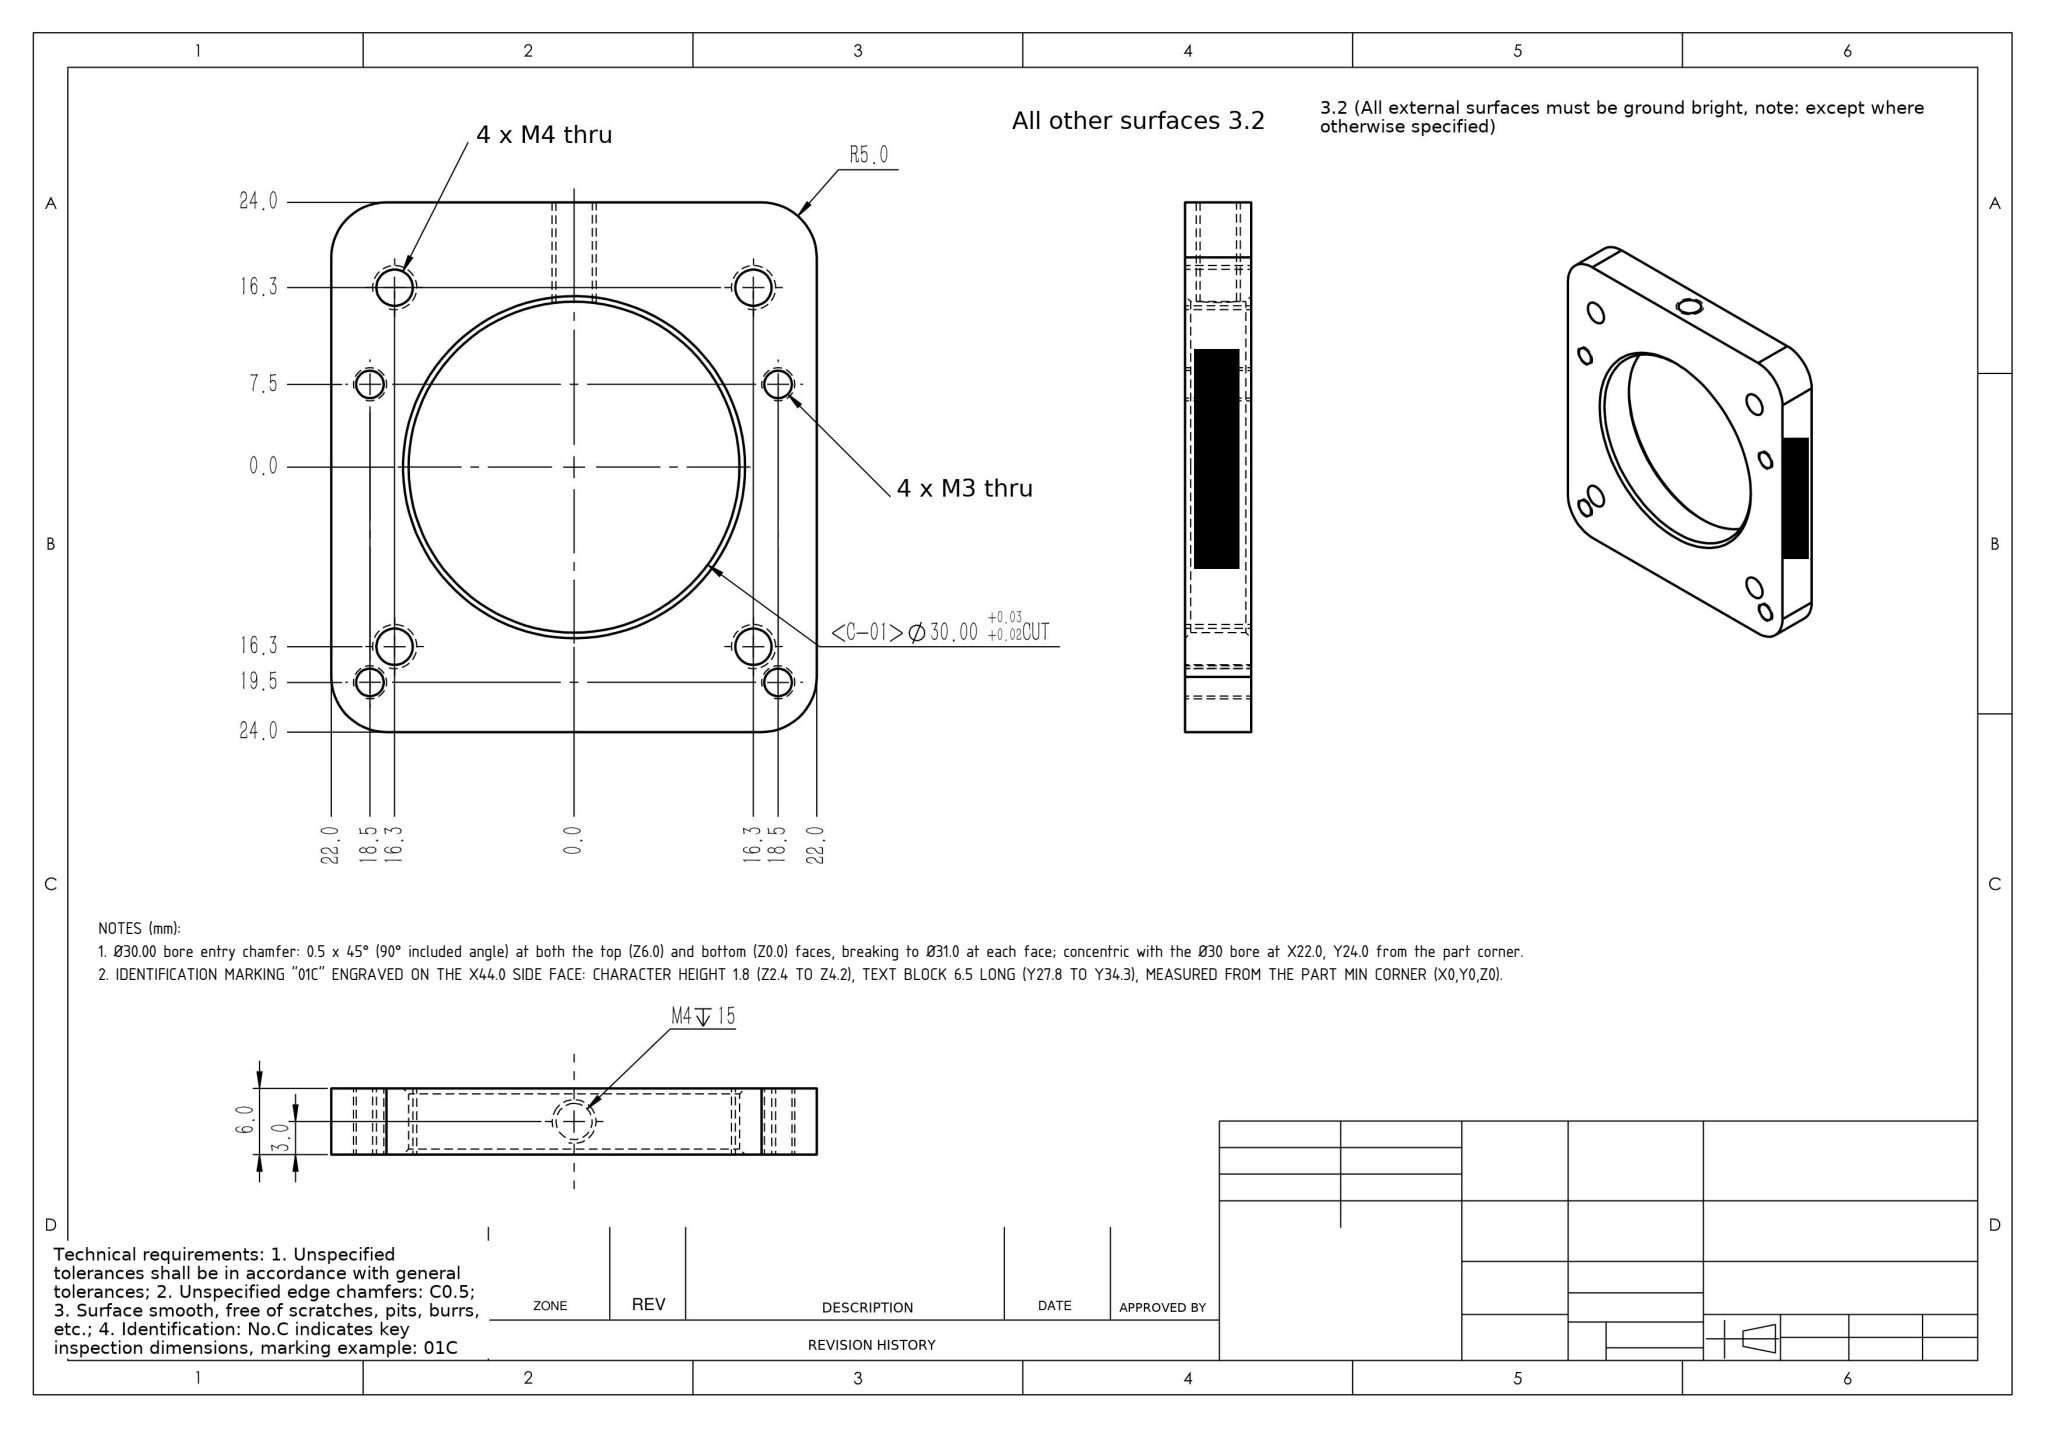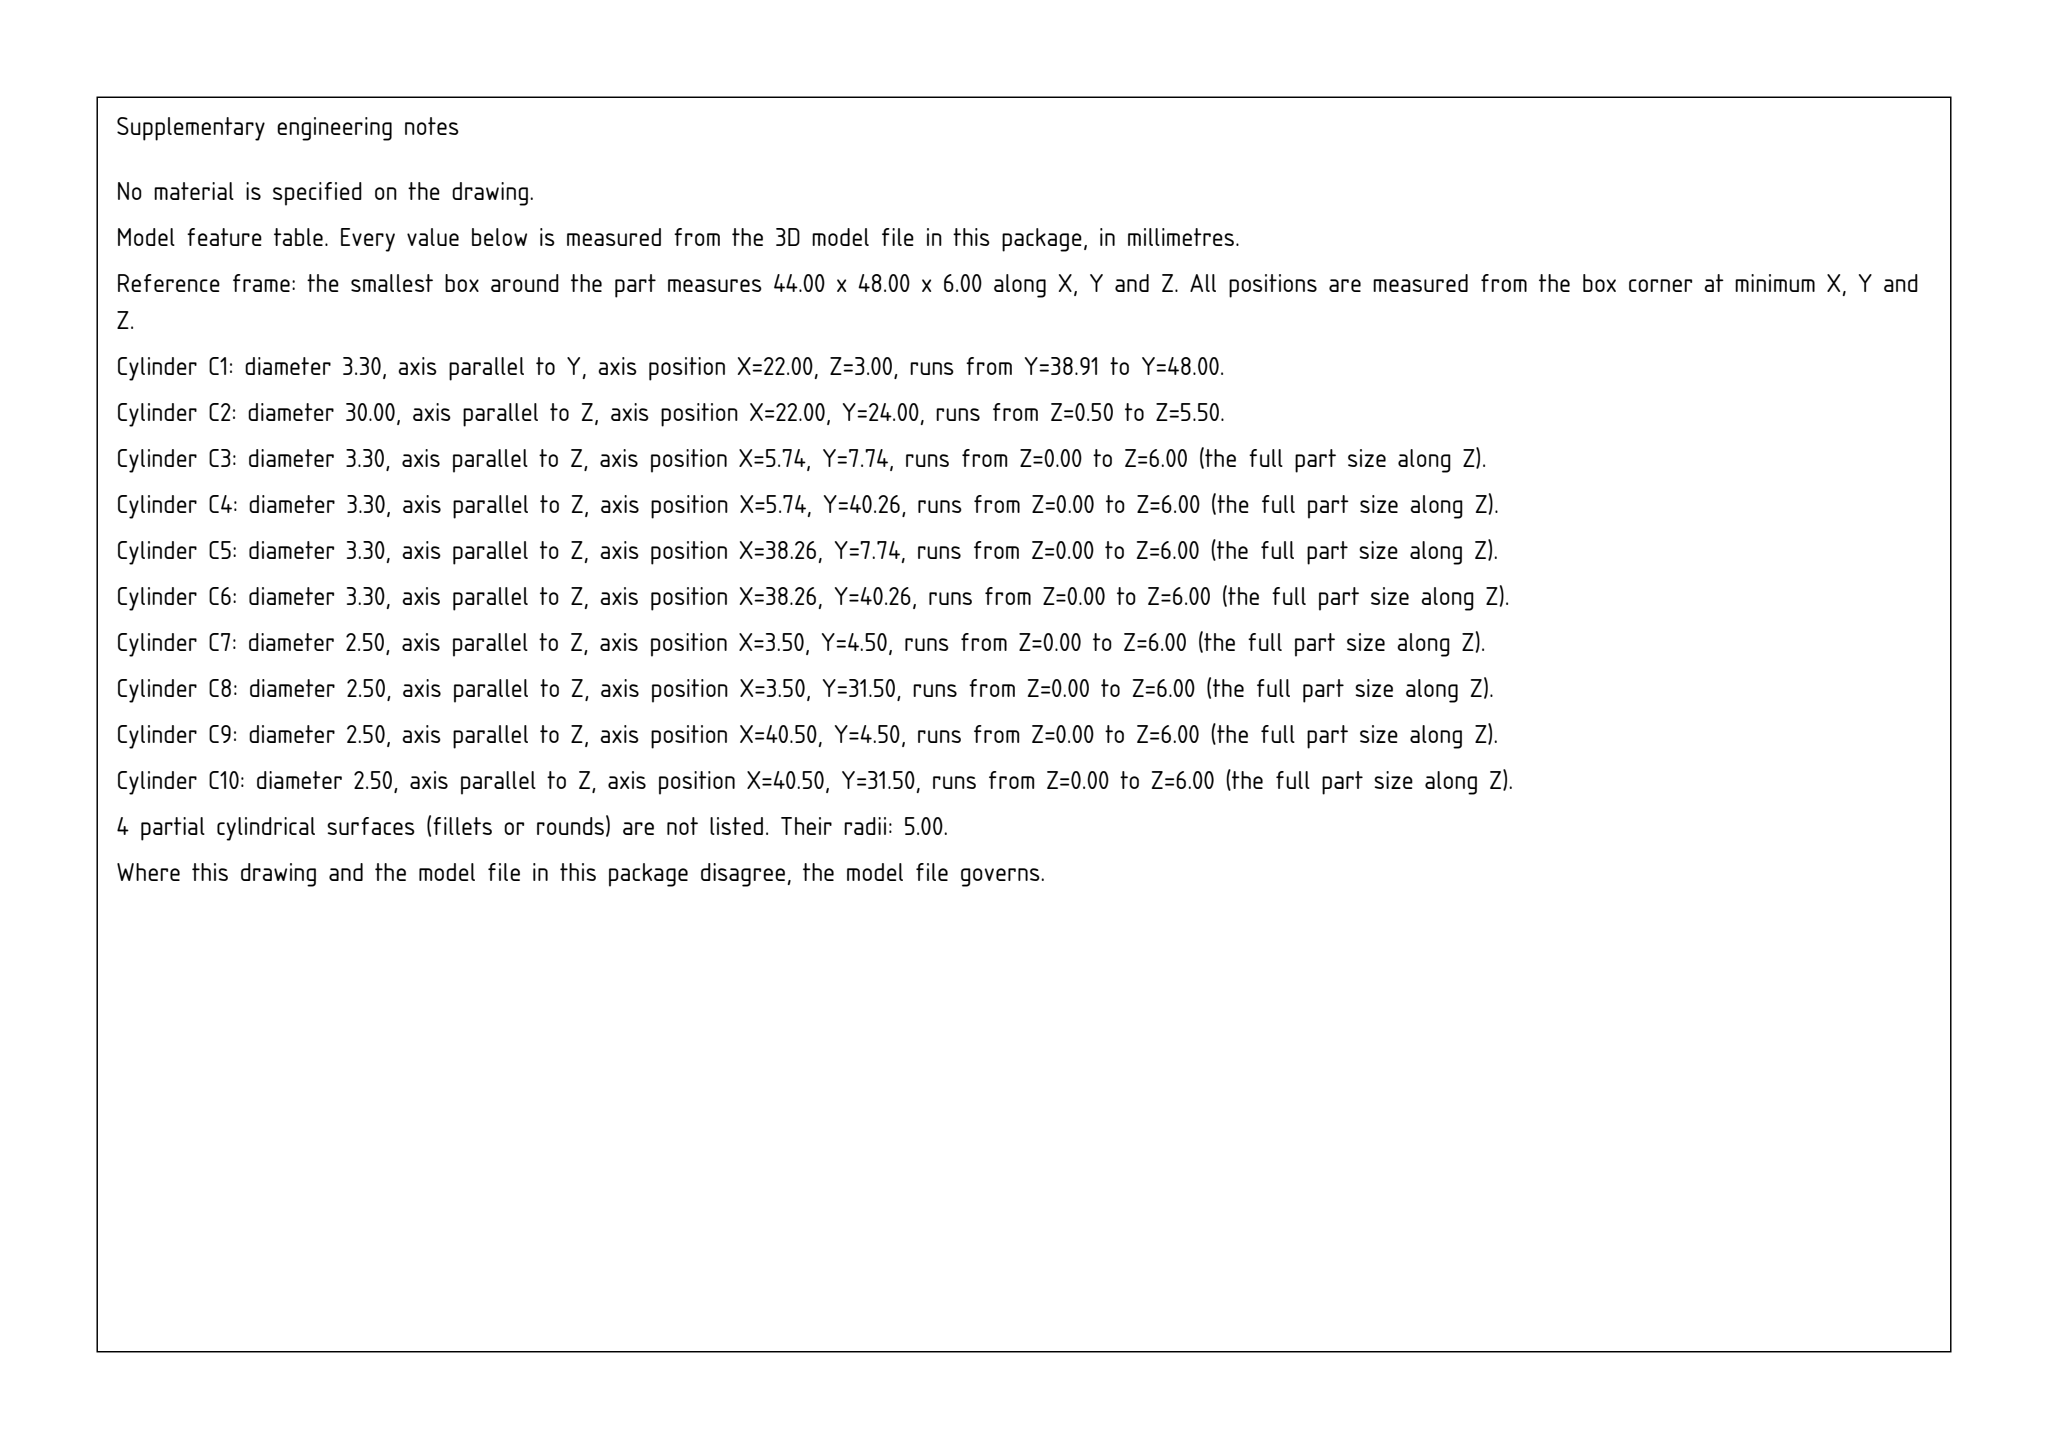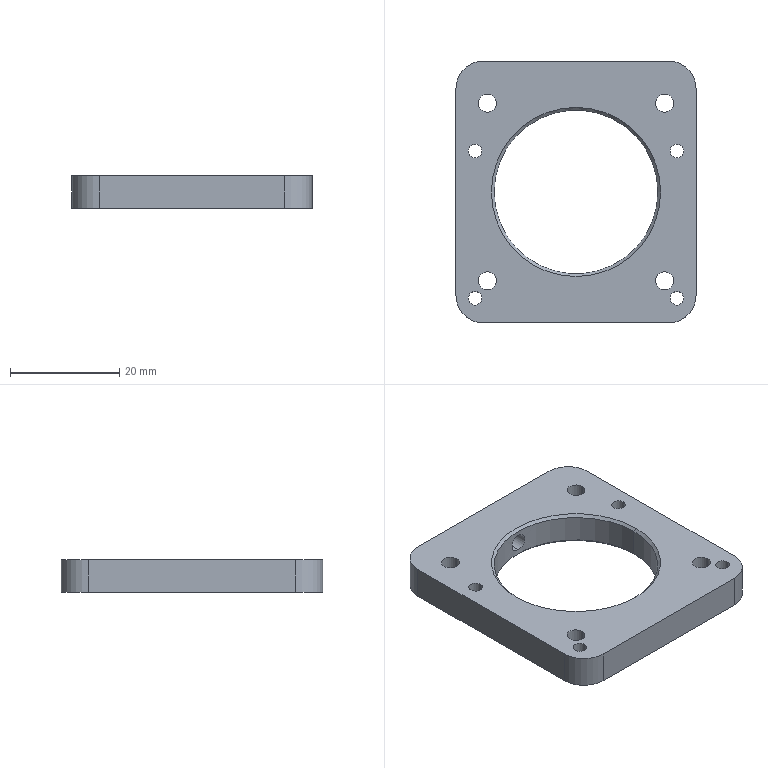Part | SolidWorks | mm | 1 solid | 43 faces | box 44 x 48 x 6 mm | volume 7878 mm3 | cylinder 24 | plane 15 | cone 4 | commonest cylinder face diameters 3.3 x10 2.5 x8 10 x4 30 x2
Drawing notes:
Ø30.00 bore entry chamfer: 0.5 x 45° (90° included angle) at both the top (Z6.0) and bottom (Z0.0) faces, breaking to Ø31.0 at each face; concentric with the Ø30 bore at X22.0, Y24.0 from the part corner. | from the solid: cones[included_angle 90.0, ref_dia 30.0/31.0, bbox_from (6.5,24.0,5.5) and (6.5,8.5,0.0), size z 0.5] together with cylinder hole/bore dia 30.0 axis z at [22.0,24.0] from 0.5 to 5.5
IDENTIFICATION MARKING "01C" ENGRAVED ON THE X44.0 SIDE FACE: CHARACTER HEIGHT 1.8 (Z2.4 TO Z4.2), TEXT BLOCK 6.5 LONG (Y27.8 TO Y34.3), MEASURED FROM THE PART MIN CORNER (X0,Y0,Z0). | from the solid: axis_planes normal x at offset 44.0: group of small glyph faces with extents y 27.8-34.3, z 2.4-4.2, lying on the x=44.0 side face (bbox 44 x 48 x 6)